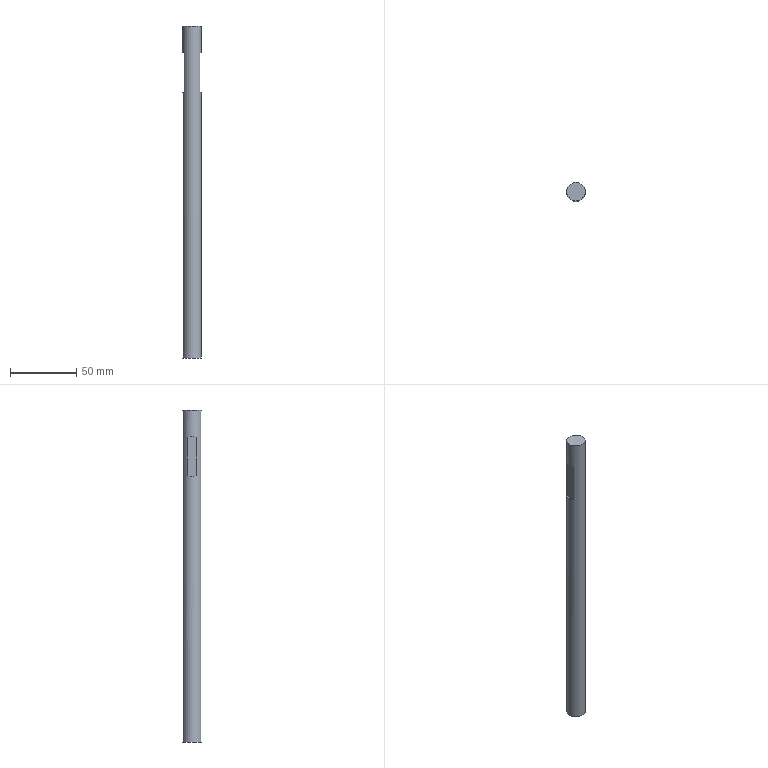Component | NX | GUIDE_ROD | 1 solid | 9 faces | box 14 x 14 x 250 mm | volume 38192 mm3 | plane 8 | cylinder 1 | commonest cylinder face diameters 14 x1
STEP:
#1=CARTESIAN_POINT('',(0.,0.,0.));
#2=DIRECTION('',(0.,0.,1.));
#3=DIRECTION('',(1.,0.,0.));
#4=AXIS2_PLACEMENT_3D('',#1,#2,#3);
#5=CARTESIAN_POINT('',(47.594,312.462,359.983));
#6=VERTEX_POINT('',#5);
#7=CARTESIAN_POINT('',(40.594,312.462,359.983));
#8=DIRECTION('',(0.,0.,1.));
#9=DIRECTION('',(1.,0.,0.));
#10=AXIS2_PLACEMENT_3D('',#7,#8,#9);
#11=CIRCLE('',#10,7.);
#12=CARTESIAN_POINT('',(40.594,312.462,359.983));
#13=DIRECTION('',(0.,0.,-1.));
#14=DIRECTION('',(-1.,0.,0.));
#15=AXIS2_PLACEMENT_3D('',#12,#13,#14);
#16=CYLINDRICAL_SURFACE('',#15,7.);
#17=CARTESIAN_POINT('',(9.425,0.));
#18=DIRECTION('',(-1.,0.));
#19=VECTOR('',#18,1.);
#20=LINE('',#17,#19);
#21=(GEOMETRIC_REPRESENTATION_CONTEXT(2)PARAMETRIC_REPRESENTATION_CONTEXT()REPRESENTATION_CONTEXT('',''));
#22=DEFINITIONAL_REPRESENTATION('',(#20),#21);
#23=PCURVE('',#16,#22);
#24=CARTESIAN_POINT('',(40.594,312.462,359.983));
#25=DIRECTION('',(0.,0.,1.));
#26=DIRECTION('',(1.,0.,0.));
#27=AXIS2_PLACEMENT_3D('',#24,#25,#26);
#28=PLANE('',#27);
#29=CARTESIAN_POINT('',(0.,0.));
#30=DIRECTION('',(1.,0.));
#31=AXIS2_PLACEMENT_2D('',#29,#30);
#32=CIRCLE('',#31,7.);
#33=(GEOMETRIC_REPRESENTATION_CONTEXT(2)PARAMETRIC_REPRESENTATION_CONTEXT()REPRESENTATION_CONTEXT('',''));
#34=DEFINITIONAL_REPRESENTATION('',(#32),#33);
#35=PCURVE('',#28,#34);
#36=SURFACE_CURVE('',#11,(#23,#35),.PCURVE_S1.);
#37=EDGE_CURVE('',#6,#6,#36,.T.);
#38=ORIENTED_EDGE('',*,*,#37,.F.);
#39=CARTESIAN_POINT('',(47.594,312.462,339.983));
#40=VERTEX_POINT('',#39);
#41=CARTESIAN_POINT('',(47.594,312.462,359.983));
#42=CARTESIAN_POINT('',(47.594,312.462,339.983));
#43=B_SPLINE_CURVE_WITH_KNOTS('',1,(#41,#42),.UNSPECIFIED.,.F.,.F.,(2,2),(0.,20.),.PIECEWISE_BEZIER_KNOTS.);
#44=CARTESIAN_POINT('',(9.425,0.));
#45=DIRECTION('',(0.,1.));
#46=VECTOR('',#45,1.);
#47=LINE('',#44,#46);
#48=(GEOMETRIC_REPRESENTATION_CONTEXT(2)PARAMETRIC_REPRESENTATION_CONTEXT()REPRESENTATION_CONTEXT('',''));
#49=DEFINITIONAL_REPRESENTATION('',(#47),#48);
#50=PCURVE('',#16,#49);
#51=CARTESIAN_POINT('',(3.142,0.));
#52=DIRECTION('',(0.,1.));
#53=VECTOR('',#52,1.);
#54=LINE('',#51,#53);
#55=(GEOMETRIC_REPRESENTATION_CONTEXT(2)PARAMETRIC_REPRESENTATION_CONTEXT()REPRESENTATION_CONTEXT('',''));
#56=DEFINITIONAL_REPRESENTATION('',(#54),#55);
#57=PCURVE('',#16,#56);
#58=SEAM_CURVE('',#43,(#50,#57),.PCURVE_S1.);
#59=EDGE_CURVE('',#6,#40,#58,.T.);
#60=ORIENTED_EDGE('',*,*,#59,.T.);
#61=CARTESIAN_POINT('',(46.594,316.067,339.983));
#62=VERTEX_POINT('',#61);
#63=CARTESIAN_POINT('',(40.594,312.462,339.983));
#64=DIRECTION('',(0.,0.,-1.));
#65=DIRECTION('',(-1.,0.,0.));
#66=AXIS2_PLACEMENT_3D('',#63,#64,#65);
#67=CIRCLE('',#66,7.);
#68=CARTESIAN_POINT('',(6.283,20.));
#69=DIRECTION('',(1.,0.));
#70=VECTOR('',#69,1.);
#71=LINE('',#68,#70);
#72=(GEOMETRIC_REPRESENTATION_CONTEXT(2)PARAMETRIC_REPRESENTATION_CONTEXT()REPRESENTATION_CONTEXT('',''));
#73=DEFINITIONAL_REPRESENTATION('',(#71),#72);
#74=PCURVE('',#16,#73);
#75=CARTESIAN_POINT('',(61.594,62.462,339.983));
#76=DIRECTION('',(0.,0.,-1.));
#77=DIRECTION('',(-1.,0.,0.));
#78=AXIS2_PLACEMENT_3D('',#75,#76,#77);
#79=PLANE('',#78);
#80=CARTESIAN_POINT('',(21.,250.));
#81=DIRECTION('',(1.,0.));
#82=AXIS2_PLACEMENT_2D('',#80,#81);
#83=CIRCLE('',#82,7.);
#84=(GEOMETRIC_REPRESENTATION_CONTEXT(2)PARAMETRIC_REPRESENTATION_CONTEXT()REPRESENTATION_CONTEXT('',''));
#85=DEFINITIONAL_REPRESENTATION('',(#83),#84);
#86=PCURVE('',#79,#85);
#87=SURFACE_CURVE('',#67,(#74,#86),.PCURVE_S1.);
#88=EDGE_CURVE('',#62,#40,#87,.T.);
#89=ORIENTED_EDGE('',*,*,#88,.F.);
#90=CARTESIAN_POINT('',(46.594,316.067,309.983));
#91=VERTEX_POINT('',#90);
#92=CARTESIAN_POINT('',(46.594,316.067,359.983));
#93=DIRECTION('',(0.,0.,1.));
#94=VECTOR('',#93,1.);
#95=LINE('',#92,#94);
#96=CARTESIAN_POINT('',(8.884,0.));
#97=DIRECTION('',(0.,-1.));
#98=VECTOR('',#97,1.);
#99=LINE('',#96,#98);
#100=(GEOMETRIC_REPRESENTATION_CONTEXT(2)PARAMETRIC_REPRESENTATION_CONTEXT()REPRESENTATION_CONTEXT('',''));
#101=DEFINITIONAL_REPRESENTATION('',(#99),#100);
#102=PCURVE('',#16,#101);
#103=CARTESIAN_POINT('',(46.594,62.462,339.983));
#104=DIRECTION('',(1.,0.,0.));
#105=DIRECTION('',(0.,0.,-1.));
#106=AXIS2_PLACEMENT_3D('',#103,#104,#105);
#107=PLANE('',#106);
#108=CARTESIAN_POINT('',(-20.,253.606));
#109=DIRECTION('',(-1.,0.));
#110=VECTOR('',#109,1.);
#111=LINE('',#108,#110);
#112=(GEOMETRIC_REPRESENTATION_CONTEXT(2)PARAMETRIC_REPRESENTATION_CONTEXT()REPRESENTATION_CONTEXT('',''));
#113=DEFINITIONAL_REPRESENTATION('',(#111),#112);
#114=PCURVE('',#107,#113);
#115=SURFACE_CURVE('',#95,(#102,#114),.PCURVE_S1.);
#116=EDGE_CURVE('',#91,#62,#115,.T.);
#117=ORIENTED_EDGE('',*,*,#116,.F.);
#118=CARTESIAN_POINT('',(47.594,312.462,309.983));
#119=VERTEX_POINT('',#118);
#120=CARTESIAN_POINT('',(40.594,312.462,309.983));
#121=DIRECTION('',(0.,0.,1.));
#122=DIRECTION('',(1.,0.,-0.));
#123=AXIS2_PLACEMENT_3D('',#120,#121,#122);
#124=CIRCLE('',#123,7.);
#125=CARTESIAN_POINT('',(15.708,50.));
#126=DIRECTION('',(-1.,0.));
#127=VECTOR('',#126,1.);
#128=LINE('',#125,#127);
#129=(GEOMETRIC_REPRESENTATION_CONTEXT(2)PARAMETRIC_REPRESENTATION_CONTEXT()REPRESENTATION_CONTEXT('',''));
#130=DEFINITIONAL_REPRESENTATION('',(#128),#129);
#131=PCURVE('',#16,#130);
#132=CARTESIAN_POINT('',(46.594,62.462,309.983));
#133=DIRECTION('',(0.,0.,1.));
#134=DIRECTION('',(1.,0.,-0.));
#135=AXIS2_PLACEMENT_3D('',#132,#133,#134);
#136=PLANE('',#135);
#137=CARTESIAN_POINT('',(-6.,250.));
#138=DIRECTION('',(1.,0.));
#139=AXIS2_PLACEMENT_2D('',#137,#138);
#140=CIRCLE('',#139,7.);
#141=(GEOMETRIC_REPRESENTATION_CONTEXT(2)PARAMETRIC_REPRESENTATION_CONTEXT()REPRESENTATION_CONTEXT('',''));
#142=DEFINITIONAL_REPRESENTATION('',(#140),#141);
#143=PCURVE('',#136,#142);
#144=SURFACE_CURVE('',#124,(#131,#143),.PCURVE_S1.);
#145=EDGE_CURVE('',#119,#91,#144,.T.);
#146=ORIENTED_EDGE('',*,*,#145,.F.);
#147=CARTESIAN_POINT('',(47.594,312.462,109.983));
#148=VERTEX_POINT('',#147);
#149=CARTESIAN_POINT('',(47.594,312.462,309.983));
#150=CARTESIAN_POINT('',(47.594,312.462,109.983));
#151=B_SPLINE_CURVE_WITH_KNOTS('',1,(#149,#150),.UNSPECIFIED.,.F.,.F.,(2,2),(50.,250.),.PIECEWISE_BEZIER_KNOTS.);
#152=CARTESIAN_POINT('',(9.425,0.));
#153=DIRECTION('',(0.,1.));
#154=VECTOR('',#153,1.);
#155=LINE('',#152,#154);
#156=(GEOMETRIC_REPRESENTATION_CONTEXT(2)PARAMETRIC_REPRESENTATION_CONTEXT()REPRESENTATION_CONTEXT('',''));
#157=DEFINITIONAL_REPRESENTATION('',(#155),#156);
#158=PCURVE('',#16,#157);
#159=CARTESIAN_POINT('',(3.142,0.));
#160=DIRECTION('',(0.,1.));
#161=VECTOR('',#160,1.);
#162=LINE('',#159,#161);
#163=(GEOMETRIC_REPRESENTATION_CONTEXT(2)PARAMETRIC_REPRESENTATION_CONTEXT()REPRESENTATION_CONTEXT('',''));
#164=DEFINITIONAL_REPRESENTATION('',(#162),#163);
#165=PCURVE('',#16,#164);
#166=SEAM_CURVE('',#151,(#158,#165),.PCURVE_S1.);
#167=EDGE_CURVE('',#119,#148,#166,.T.);
#168=ORIENTED_EDGE('',*,*,#167,.T.);
#169=CARTESIAN_POINT('',(40.594,312.462,109.983));
#170=DIRECTION('',(0.,0.,1.));
#171=DIRECTION('',(1.,0.,0.));
#172=AXIS2_PLACEMENT_3D('',#169,#170,#171);
#173=CIRCLE('',#172,7.);
#174=CARTESIAN_POINT('',(9.425,250.));
#175=DIRECTION('',(-1.,0.));
#176=VECTOR('',#175,1.);
#177=LINE('',#174,#176);
#178=(GEOMETRIC_REPRESENTATION_CONTEXT(2)PARAMETRIC_REPRESENTATION_CONTEXT()REPRESENTATION_CONTEXT('',''));
#179=DEFINITIONAL_REPRESENTATION('',(#177),#178);
#180=PCURVE('',#16,#179);
#181=CARTESIAN_POINT('',(40.594,312.462,109.983));
#182=DIRECTION('',(0.,0.,1.));
#183=DIRECTION('',(1.,0.,0.));
#184=AXIS2_PLACEMENT_3D('',#181,#182,#183);
#185=PLANE('',#184);
#186=CARTESIAN_POINT('',(0.,0.));
#187=DIRECTION('',(1.,0.));
#188=AXIS2_PLACEMENT_2D('',#186,#187);
#189=CIRCLE('',#188,7.);
#190=(GEOMETRIC_REPRESENTATION_CONTEXT(2)PARAMETRIC_REPRESENTATION_CONTEXT()REPRESENTATION_CONTEXT('',''));
#191=DEFINITIONAL_REPRESENTATION('',(#189),#190);
#192=PCURVE('',#185,#191);
#193=SURFACE_CURVE('',#173,(#180,#192),.PCURVE_S1.);
#194=EDGE_CURVE('',#148,#148,#193,.T.);
#195=ORIENTED_EDGE('',*,*,#194,.T.);
#196=ORIENTED_EDGE('',*,*,#167,.F.);
#197=CARTESIAN_POINT('',(46.594,308.856,309.983));
#198=VERTEX_POINT('',#197);
#199=CARTESIAN_POINT('',(40.594,312.462,309.983));
#200=DIRECTION('',(0.,0.,1.));
#201=DIRECTION('',(1.,0.,-0.));
#202=AXIS2_PLACEMENT_3D('',#199,#200,#201);
#203=CIRCLE('',#202,7.);
#204=CARTESIAN_POINT('',(9.425,50.));
#205=DIRECTION('',(-1.,0.));
#206=VECTOR('',#205,1.);
#207=LINE('',#204,#206);
#208=(GEOMETRIC_REPRESENTATION_CONTEXT(2)PARAMETRIC_REPRESENTATION_CONTEXT()REPRESENTATION_CONTEXT('',''));
#209=DEFINITIONAL_REPRESENTATION('',(#207),#208);
#210=PCURVE('',#16,#209);
#211=CARTESIAN_POINT('',(-6.,250.));
#212=DIRECTION('',(1.,0.));
#213=AXIS2_PLACEMENT_2D('',#211,#212);
#214=CIRCLE('',#213,7.);
#215=(GEOMETRIC_REPRESENTATION_CONTEXT(2)PARAMETRIC_REPRESENTATION_CONTEXT()REPRESENTATION_CONTEXT('',''));
#216=DEFINITIONAL_REPRESENTATION('',(#214),#215);
#217=PCURVE('',#136,#216);
#218=SURFACE_CURVE('',#203,(#210,#217),.PCURVE_S1.);
#219=EDGE_CURVE('',#198,#119,#218,.T.);
#220=ORIENTED_EDGE('',*,*,#219,.F.);
#221=CARTESIAN_POINT('',(46.594,308.856,339.983));
#222=VERTEX_POINT('',#221);
#223=CARTESIAN_POINT('',(46.594,308.856,359.983));
#224=DIRECTION('',(0.,0.,-1.));
#225=VECTOR('',#224,1.);
#226=LINE('',#223,#225);
#227=CARTESIAN_POINT('',(3.683,0.));
#228=DIRECTION('',(0.,1.));
#229=VECTOR('',#228,1.);
#230=LINE('',#227,#229);
#231=(GEOMETRIC_REPRESENTATION_CONTEXT(2)PARAMETRIC_REPRESENTATION_CONTEXT()REPRESENTATION_CONTEXT('',''));
#232=DEFINITIONAL_REPRESENTATION('',(#230),#231);
#233=PCURVE('',#16,#232);
#234=CARTESIAN_POINT('',(-20.,246.394));
#235=DIRECTION('',(1.,0.));
#236=VECTOR('',#235,1.);
#237=LINE('',#234,#236);
#238=(GEOMETRIC_REPRESENTATION_CONTEXT(2)PARAMETRIC_REPRESENTATION_CONTEXT()REPRESENTATION_CONTEXT('',''));
#239=DEFINITIONAL_REPRESENTATION('',(#237),#238);
#240=PCURVE('',#107,#239);
#241=SURFACE_CURVE('',#226,(#233,#240),.PCURVE_S1.);
#242=EDGE_CURVE('',#222,#198,#241,.T.);
#243=ORIENTED_EDGE('',*,*,#242,.F.);
#244=CARTESIAN_POINT('',(40.594,312.462,339.983));
#245=DIRECTION('',(0.,0.,-1.));
#246=DIRECTION('',(-1.,0.,0.));
#247=AXIS2_PLACEMENT_3D('',#244,#245,#246);
#248=CIRCLE('',#247,7.);
#249=CARTESIAN_POINT('',(-0.,20.));
#250=DIRECTION('',(1.,0.));
#251=VECTOR('',#250,1.);
#252=LINE('',#249,#251);
#253=(GEOMETRIC_REPRESENTATION_CONTEXT(2)PARAMETRIC_REPRESENTATION_CONTEXT()REPRESENTATION_CONTEXT('',''));
#254=DEFINITIONAL_REPRESENTATION('',(#252),#253);
#255=PCURVE('',#16,#254);
#256=CARTESIAN_POINT('',(21.,250.));
#257=DIRECTION('',(1.,0.));
#258=AXIS2_PLACEMENT_2D('',#256,#257);
#259=CIRCLE('',#258,7.);
#260=(GEOMETRIC_REPRESENTATION_CONTEXT(2)PARAMETRIC_REPRESENTATION_CONTEXT()REPRESENTATION_CONTEXT('',''));
#261=DEFINITIONAL_REPRESENTATION('',(#259),#260);
#262=PCURVE('',#79,#261);
#263=SURFACE_CURVE('',#248,(#255,#262),.PCURVE_S1.);
#264=EDGE_CURVE('',#40,#222,#263,.T.);
#265=ORIENTED_EDGE('',*,*,#264,.F.);
#266=ORIENTED_EDGE('',*,*,#59,.F.);
#267=EDGE_LOOP('',(#38,#60,#89,#117,#146,#168,#195,#196,#220,#243,#265,#266));
#268=FACE_BOUND('',#267,.T.);
#269=CARTESIAN_POINT('',(34.594,316.067,309.983));
#270=VERTEX_POINT('',#269);
#271=CARTESIAN_POINT('',(34.594,308.856,309.983));
#272=VERTEX_POINT('',#271);
#273=CARTESIAN_POINT('',(40.594,312.462,309.983));
#274=DIRECTION('',(-0.,0.,1.));
#275=DIRECTION('',(1.,0.,0.));
#276=AXIS2_PLACEMENT_3D('',#273,#274,#275);
#277=CIRCLE('',#276,7.);
#278=CARTESIAN_POINT('',(9.425,50.));
#279=DIRECTION('',(-1.,0.));
#280=VECTOR('',#279,1.);
#281=LINE('',#278,#280);
#282=(GEOMETRIC_REPRESENTATION_CONTEXT(2)PARAMETRIC_REPRESENTATION_CONTEXT()REPRESENTATION_CONTEXT('',''));
#283=DEFINITIONAL_REPRESENTATION('',(#281),#282);
#284=PCURVE('',#16,#283);
#285=CARTESIAN_POINT('',(25.594,62.462,309.983));
#286=DIRECTION('',(-0.,0.,1.));
#287=DIRECTION('',(1.,0.,0.));
#288=AXIS2_PLACEMENT_3D('',#285,#286,#287);
#289=PLANE('',#288);
#290=CARTESIAN_POINT('',(15.,250.));
#291=DIRECTION('',(1.,0.));
#292=AXIS2_PLACEMENT_2D('',#290,#291);
#293=CIRCLE('',#292,7.);
#294=(GEOMETRIC_REPRESENTATION_CONTEXT(2)PARAMETRIC_REPRESENTATION_CONTEXT()REPRESENTATION_CONTEXT('',''));
#295=DEFINITIONAL_REPRESENTATION('',(#293),#294);
#296=PCURVE('',#289,#295);
#297=SURFACE_CURVE('',#277,(#284,#296),.PCURVE_S1.);
#298=EDGE_CURVE('',#270,#272,#297,.T.);
#299=ORIENTED_EDGE('',*,*,#298,.F.);
#300=CARTESIAN_POINT('',(34.594,316.067,339.983));
#301=VERTEX_POINT('',#300);
#302=CARTESIAN_POINT('',(34.594,316.067,359.983));
#303=DIRECTION('',(0.,0.,-1.));
#304=VECTOR('',#303,1.);
#305=LINE('',#302,#304);
#306=CARTESIAN_POINT('',(6.824,0.));
#307=DIRECTION('',(0.,1.));
#308=VECTOR('',#307,1.);
#309=LINE('',#306,#308);
#310=(GEOMETRIC_REPRESENTATION_CONTEXT(2)PARAMETRIC_REPRESENTATION_CONTEXT()REPRESENTATION_CONTEXT('',''));
#311=DEFINITIONAL_REPRESENTATION('',(#309),#310);
#312=PCURVE('',#16,#311);
#313=CARTESIAN_POINT('',(34.594,62.462,309.983));
#314=DIRECTION('',(-1.,0.,-0.));
#315=DIRECTION('',(-0.,0.,1.));
#316=AXIS2_PLACEMENT_3D('',#313,#314,#315);
#317=PLANE('',#316);
#318=CARTESIAN_POINT('',(50.,253.606));
#319=DIRECTION('',(-1.,0.));
#320=VECTOR('',#319,1.);
#321=LINE('',#318,#320);
#322=(GEOMETRIC_REPRESENTATION_CONTEXT(2)PARAMETRIC_REPRESENTATION_CONTEXT()REPRESENTATION_CONTEXT('',''));
#323=DEFINITIONAL_REPRESENTATION('',(#321),#322);
#324=PCURVE('',#317,#323);
#325=SURFACE_CURVE('',#305,(#312,#324),.PCURVE_S1.);
#326=EDGE_CURVE('',#301,#270,#325,.T.);
#327=ORIENTED_EDGE('',*,*,#326,.F.);
#328=CARTESIAN_POINT('',(34.594,308.856,339.983));
#329=VERTEX_POINT('',#328);
#330=CARTESIAN_POINT('',(40.594,312.462,339.983));
#331=DIRECTION('',(0.,0.,-1.));
#332=DIRECTION('',(-1.,0.,0.));
#333=AXIS2_PLACEMENT_3D('',#330,#331,#332);
#334=CIRCLE('',#333,7.);
#335=CARTESIAN_POINT('',(0.,20.));
#336=DIRECTION('',(1.,0.));
#337=VECTOR('',#336,1.);
#338=LINE('',#335,#337);
#339=(GEOMETRIC_REPRESENTATION_CONTEXT(2)PARAMETRIC_REPRESENTATION_CONTEXT()REPRESENTATION_CONTEXT('',''));
#340=DEFINITIONAL_REPRESENTATION('',(#338),#339);
#341=PCURVE('',#16,#340);
#342=CARTESIAN_POINT('',(34.594,62.462,339.983));
#343=DIRECTION('',(0.,0.,-1.));
#344=DIRECTION('',(-1.,0.,0.));
#345=AXIS2_PLACEMENT_3D('',#342,#343,#344);
#346=PLANE('',#345);
#347=CARTESIAN_POINT('',(-6.,250.));
#348=DIRECTION('',(1.,0.));
#349=AXIS2_PLACEMENT_2D('',#347,#348);
#350=CIRCLE('',#349,7.);
#351=(GEOMETRIC_REPRESENTATION_CONTEXT(2)PARAMETRIC_REPRESENTATION_CONTEXT()REPRESENTATION_CONTEXT('',''));
#352=DEFINITIONAL_REPRESENTATION('',(#350),#351);
#353=PCURVE('',#346,#352);
#354=SURFACE_CURVE('',#334,(#341,#353),.PCURVE_S1.);
#355=EDGE_CURVE('',#329,#301,#354,.T.);
#356=ORIENTED_EDGE('',*,*,#355,.F.);
#357=CARTESIAN_POINT('',(34.594,308.856,359.983));
#358=DIRECTION('',(0.,0.,1.));
#359=VECTOR('',#358,1.);
#360=LINE('',#357,#359);
#361=CARTESIAN_POINT('',(5.742,0.));
#362=DIRECTION('',(0.,-1.));
#363=VECTOR('',#362,1.);
#364=LINE('',#361,#363);
#365=(GEOMETRIC_REPRESENTATION_CONTEXT(2)PARAMETRIC_REPRESENTATION_CONTEXT()REPRESENTATION_CONTEXT('',''));
#366=DEFINITIONAL_REPRESENTATION('',(#364),#365);
#367=PCURVE('',#16,#366);
#368=CARTESIAN_POINT('',(50.,246.394));
#369=DIRECTION('',(1.,0.));
#370=VECTOR('',#369,1.);
#371=LINE('',#368,#370);
#372=(GEOMETRIC_REPRESENTATION_CONTEXT(2)PARAMETRIC_REPRESENTATION_CONTEXT()REPRESENTATION_CONTEXT('',''));
#373=DEFINITIONAL_REPRESENTATION('',(#371),#372);
#374=PCURVE('',#317,#373);
#375=SURFACE_CURVE('',#360,(#367,#374),.PCURVE_S1.);
#376=EDGE_CURVE('',#272,#329,#375,.T.);
#377=ORIENTED_EDGE('',*,*,#376,.F.);
#378=EDGE_LOOP('',(#299,#327,#356,#377));
#379=FACE_BOUND('',#378,.T.);
#380=ADVANCED_FACE('',(#268,#379),#16,.T.);
#381=ORIENTED_EDGE('',*,*,#37,.T.);
#382=EDGE_LOOP('',(#381));
#383=FACE_BOUND('',#382,.T.);
#384=ADVANCED_FACE('',(#383),#28,.T.);
#385=ORIENTED_EDGE('',*,*,#194,.F.);
#386=EDGE_LOOP('',(#385));
#387=FACE_BOUND('',#386,.T.);
#388=ADVANCED_FACE('',(#387),#185,.F.);
#389=ORIENTED_EDGE('',*,*,#298,.T.);
#390=CARTESIAN_POINT('',(34.594,62.462,309.983));
#391=DIRECTION('',(0.,-1.,0.));
#392=VECTOR('',#391,1.);
#393=LINE('',#390,#392);
#394=CARTESIAN_POINT('',(9.,0.));
#395=DIRECTION('',(0.,-1.));
#396=VECTOR('',#395,1.);
#397=LINE('',#394,#396);
#398=(GEOMETRIC_REPRESENTATION_CONTEXT(2)PARAMETRIC_REPRESENTATION_CONTEXT()REPRESENTATION_CONTEXT('',''));
#399=DEFINITIONAL_REPRESENTATION('',(#397),#398);
#400=PCURVE('',#289,#399);
#401=CARTESIAN_POINT('',(0.,0.));
#402=DIRECTION('',(0.,-1.));
#403=VECTOR('',#402,1.);
#404=LINE('',#401,#403);
#405=(GEOMETRIC_REPRESENTATION_CONTEXT(2)PARAMETRIC_REPRESENTATION_CONTEXT()REPRESENTATION_CONTEXT('',''));
#406=DEFINITIONAL_REPRESENTATION('',(#404),#405);
#407=PCURVE('',#317,#406);
#408=SURFACE_CURVE('',#393,(#400,#407),.PCURVE_S1.);
#409=EDGE_CURVE('',#270,#272,#408,.T.);
#410=ORIENTED_EDGE('',*,*,#409,.F.);
#411=EDGE_LOOP('',(#389,#410));
#412=FACE_BOUND('',#411,.T.);
#413=ADVANCED_FACE('',(#412),#289,.T.);
#414=ORIENTED_EDGE('',*,*,#326,.T.);
#415=ORIENTED_EDGE('',*,*,#409,.T.);
#416=ORIENTED_EDGE('',*,*,#376,.T.);
#417=CARTESIAN_POINT('',(34.594,62.462,339.983));
#418=DIRECTION('',(0.,-1.,0.));
#419=VECTOR('',#418,1.);
#420=LINE('',#417,#419);
#421=CARTESIAN_POINT('',(30.,0.));
#422=DIRECTION('',(0.,-1.));
#423=VECTOR('',#422,1.);
#424=LINE('',#421,#423);
#425=(GEOMETRIC_REPRESENTATION_CONTEXT(2)PARAMETRIC_REPRESENTATION_CONTEXT()REPRESENTATION_CONTEXT('',''));
#426=DEFINITIONAL_REPRESENTATION('',(#424),#425);
#427=PCURVE('',#317,#426);
#428=CARTESIAN_POINT('',(0.,0.));
#429=DIRECTION('',(0.,-1.));
#430=VECTOR('',#429,1.);
#431=LINE('',#428,#430);
#432=(GEOMETRIC_REPRESENTATION_CONTEXT(2)PARAMETRIC_REPRESENTATION_CONTEXT()REPRESENTATION_CONTEXT('',''));
#433=DEFINITIONAL_REPRESENTATION('',(#431),#432);
#434=PCURVE('',#346,#433);
#435=SURFACE_CURVE('',#420,(#427,#434),.PCURVE_S1.);
#436=EDGE_CURVE('',#301,#329,#435,.T.);
#437=ORIENTED_EDGE('',*,*,#436,.F.);
#438=EDGE_LOOP('',(#414,#415,#416,#437));
#439=FACE_BOUND('',#438,.T.);
#440=ADVANCED_FACE('',(#439),#317,.T.);
#441=ORIENTED_EDGE('',*,*,#355,.T.);
#442=ORIENTED_EDGE('',*,*,#436,.T.);
#443=EDGE_LOOP('',(#441,#442));
#444=FACE_BOUND('',#443,.T.);
#445=ADVANCED_FACE('',(#444),#346,.T.);
#446=ORIENTED_EDGE('',*,*,#242,.T.);
#447=CARTESIAN_POINT('',(46.594,62.462,309.983));
#448=DIRECTION('',(0.,-1.,0.));
#449=VECTOR('',#448,1.);
#450=LINE('',#447,#449);
#451=CARTESIAN_POINT('',(30.,0.));
#452=DIRECTION('',(0.,-1.));
#453=VECTOR('',#452,1.);
#454=LINE('',#451,#453);
#455=(GEOMETRIC_REPRESENTATION_CONTEXT(2)PARAMETRIC_REPRESENTATION_CONTEXT()REPRESENTATION_CONTEXT('',''));
#456=DEFINITIONAL_REPRESENTATION('',(#454),#455);
#457=PCURVE('',#107,#456);
#458=CARTESIAN_POINT('',(0.,0.));
#459=DIRECTION('',(0.,-1.));
#460=VECTOR('',#459,1.);
#461=LINE('',#458,#460);
#462=(GEOMETRIC_REPRESENTATION_CONTEXT(2)PARAMETRIC_REPRESENTATION_CONTEXT()REPRESENTATION_CONTEXT('',''));
#463=DEFINITIONAL_REPRESENTATION('',(#461),#462);
#464=PCURVE('',#136,#463);
#465=SURFACE_CURVE('',#450,(#457,#464),.PCURVE_S1.);
#466=EDGE_CURVE('',#91,#198,#465,.T.);
#467=ORIENTED_EDGE('',*,*,#466,.F.);
#468=ORIENTED_EDGE('',*,*,#116,.T.);
#469=CARTESIAN_POINT('',(46.594,62.462,339.983));
#470=DIRECTION('',(0.,-1.,0.));
#471=VECTOR('',#470,1.);
#472=LINE('',#469,#471);
#473=CARTESIAN_POINT('',(0.,0.));
#474=DIRECTION('',(0.,-1.));
#475=VECTOR('',#474,1.);
#476=LINE('',#473,#475);
#477=(GEOMETRIC_REPRESENTATION_CONTEXT(2)PARAMETRIC_REPRESENTATION_CONTEXT()REPRESENTATION_CONTEXT('',''));
#478=DEFINITIONAL_REPRESENTATION('',(#476),#477);
#479=PCURVE('',#107,#478);
#480=CARTESIAN_POINT('',(15.,0.));
#481=DIRECTION('',(0.,-1.));
#482=VECTOR('',#481,1.);
#483=LINE('',#480,#482);
#484=(GEOMETRIC_REPRESENTATION_CONTEXT(2)PARAMETRIC_REPRESENTATION_CONTEXT()REPRESENTATION_CONTEXT('',''));
#485=DEFINITIONAL_REPRESENTATION('',(#483),#484);
#486=PCURVE('',#79,#485);
#487=SURFACE_CURVE('',#472,(#479,#486),.PCURVE_S1.);
#488=EDGE_CURVE('',#62,#222,#487,.T.);
#489=ORIENTED_EDGE('',*,*,#488,.T.);
#490=EDGE_LOOP('',(#446,#467,#468,#489));
#491=FACE_BOUND('',#490,.T.);
#492=ADVANCED_FACE('',(#491),#107,.T.);
#493=ORIENTED_EDGE('',*,*,#219,.T.);
#494=ORIENTED_EDGE('',*,*,#145,.T.);
#495=ORIENTED_EDGE('',*,*,#466,.T.);
#496=EDGE_LOOP('',(#493,#494,#495));
#497=FACE_BOUND('',#496,.T.);
#498=ADVANCED_FACE('',(#497),#136,.T.);
#499=ORIENTED_EDGE('',*,*,#88,.T.);
#500=ORIENTED_EDGE('',*,*,#264,.T.);
#501=ORIENTED_EDGE('',*,*,#488,.F.);
#502=EDGE_LOOP('',(#499,#500,#501));
#503=FACE_BOUND('',#502,.T.);
#504=ADVANCED_FACE('',(#503),#79,.T.);
#505=CLOSED_SHELL('',(#380,#384,#388,#413,#440,#445,#492,#498,#504));
#506=MANIFOLD_SOLID_BREP('',#505);
#507=(LENGTH_UNIT()NAMED_UNIT(*)SI_UNIT(.MILLI.,.METRE.));
#508=UNCERTAINTY_MEASURE_WITH_UNIT(LENGTH_MEASURE(0.000002),#507,'','');
#509=(NAMED_UNIT(*)PLANE_ANGLE_UNIT()SI_UNIT($,.RADIAN.));
#510=(NAMED_UNIT(*)SI_UNIT($,.STERADIAN.)SOLID_ANGLE_UNIT());
#511=(GEOMETRIC_REPRESENTATION_CONTEXT(3)GLOBAL_UNCERTAINTY_ASSIGNED_CONTEXT((#508))GLOBAL_UNIT_ASSIGNED_CONTEXT((#507,#509,#510))REPRESENTATION_CONTEXT('',''));
#512=ADVANCED_BREP_SHAPE_REPRESENTATION('',(#4,#506),#511);